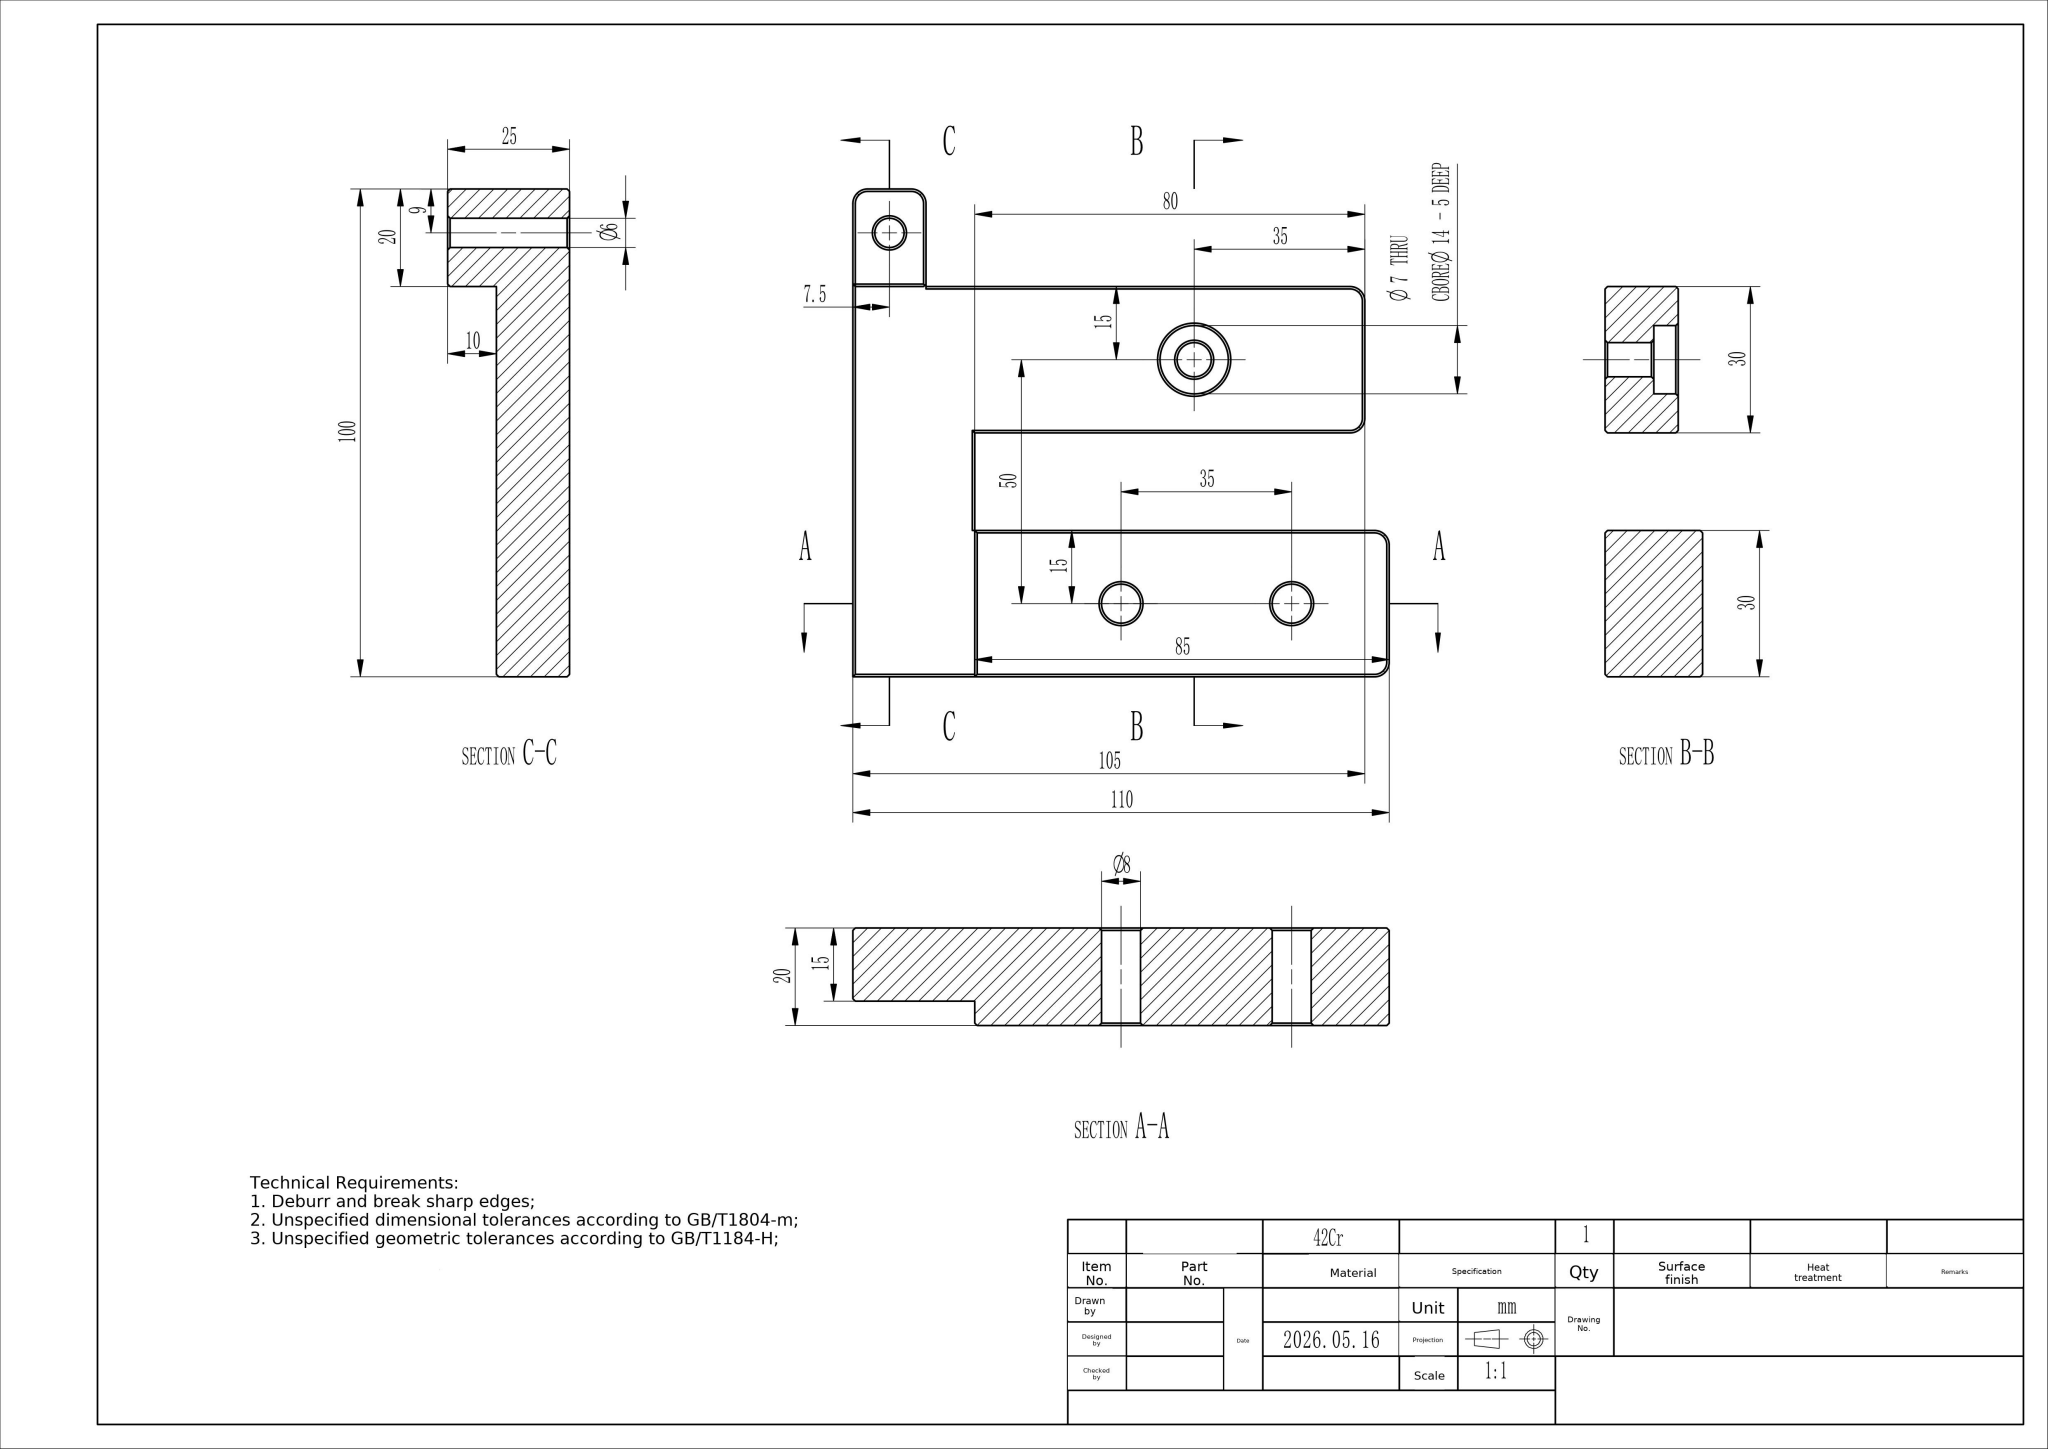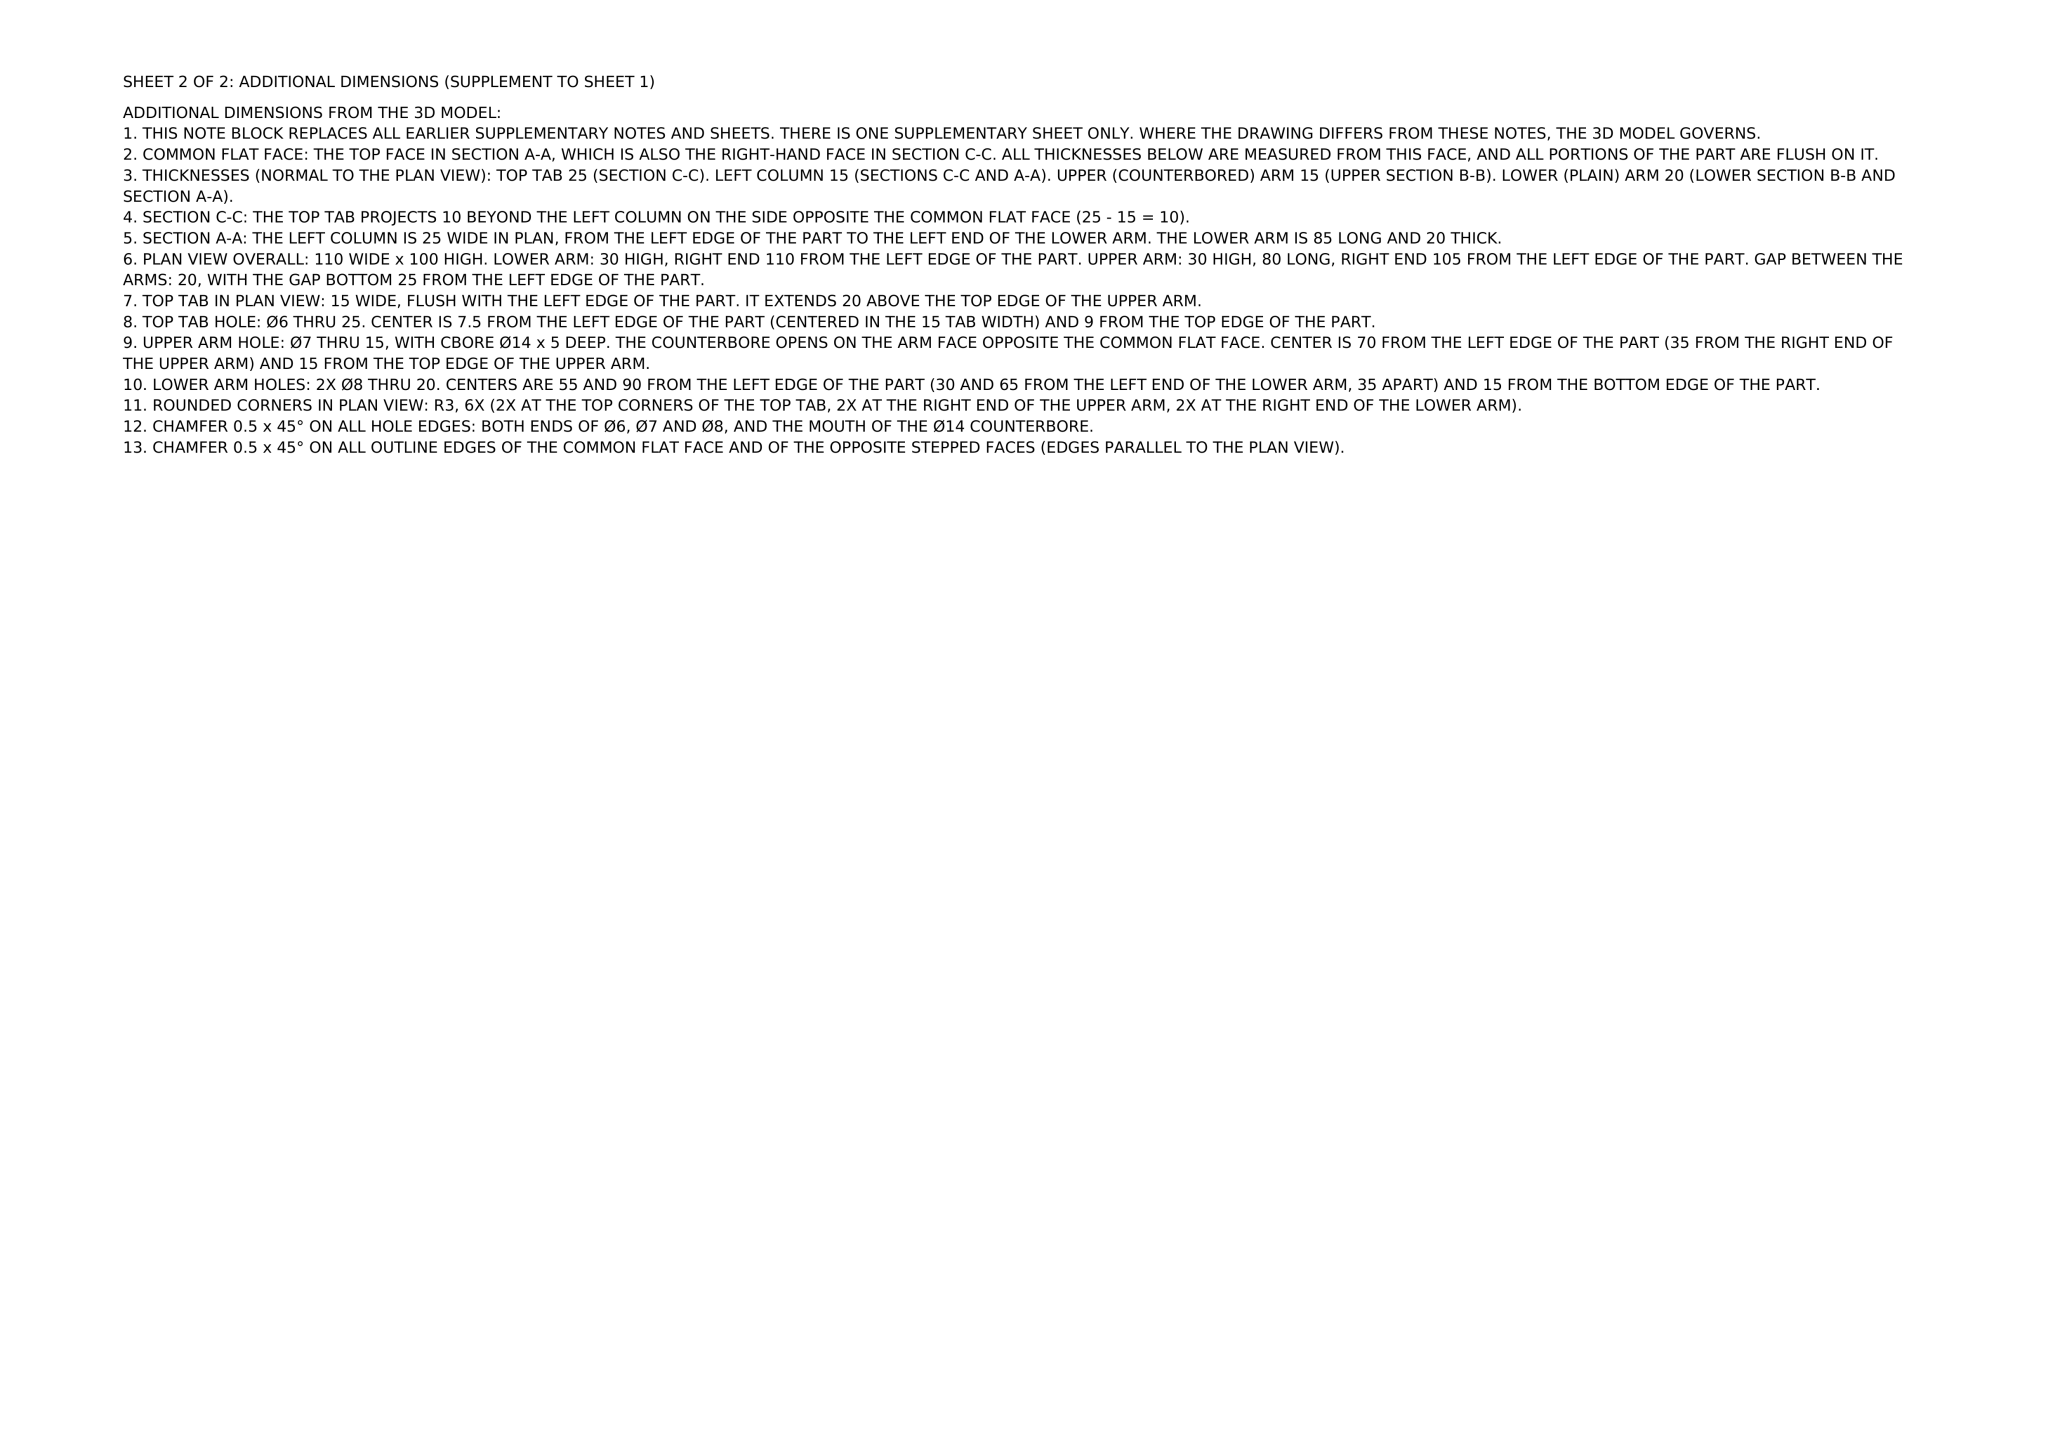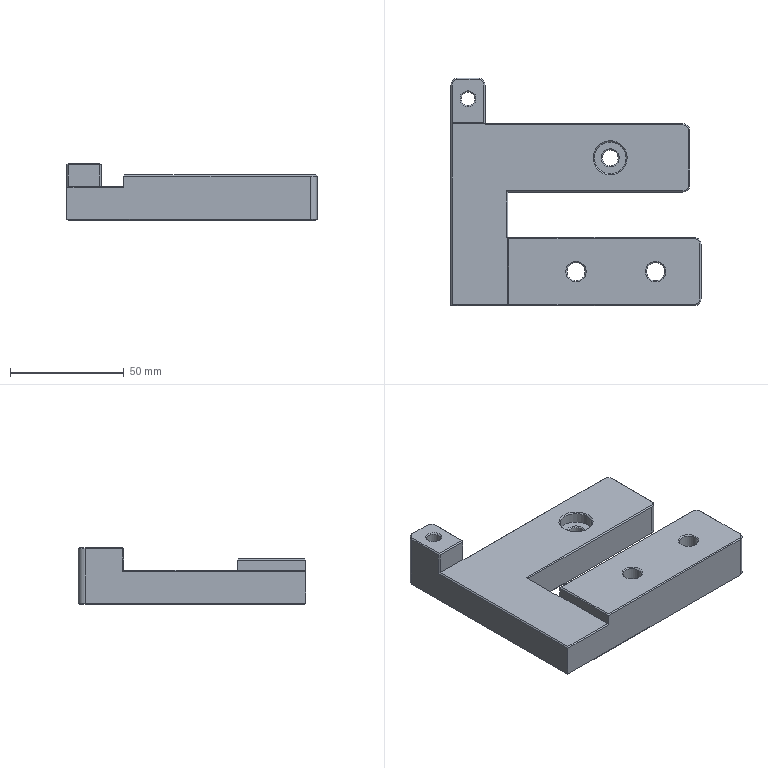Part | NX | mm | 1 solid | 76 faces | box 110 x 100 x 25 mm | volume 120216 mm3 | plane 44 | cone 21 | cylinder 11 | commonest cylinder face diameters 6 x7 8 x2 7 x1 14 x1